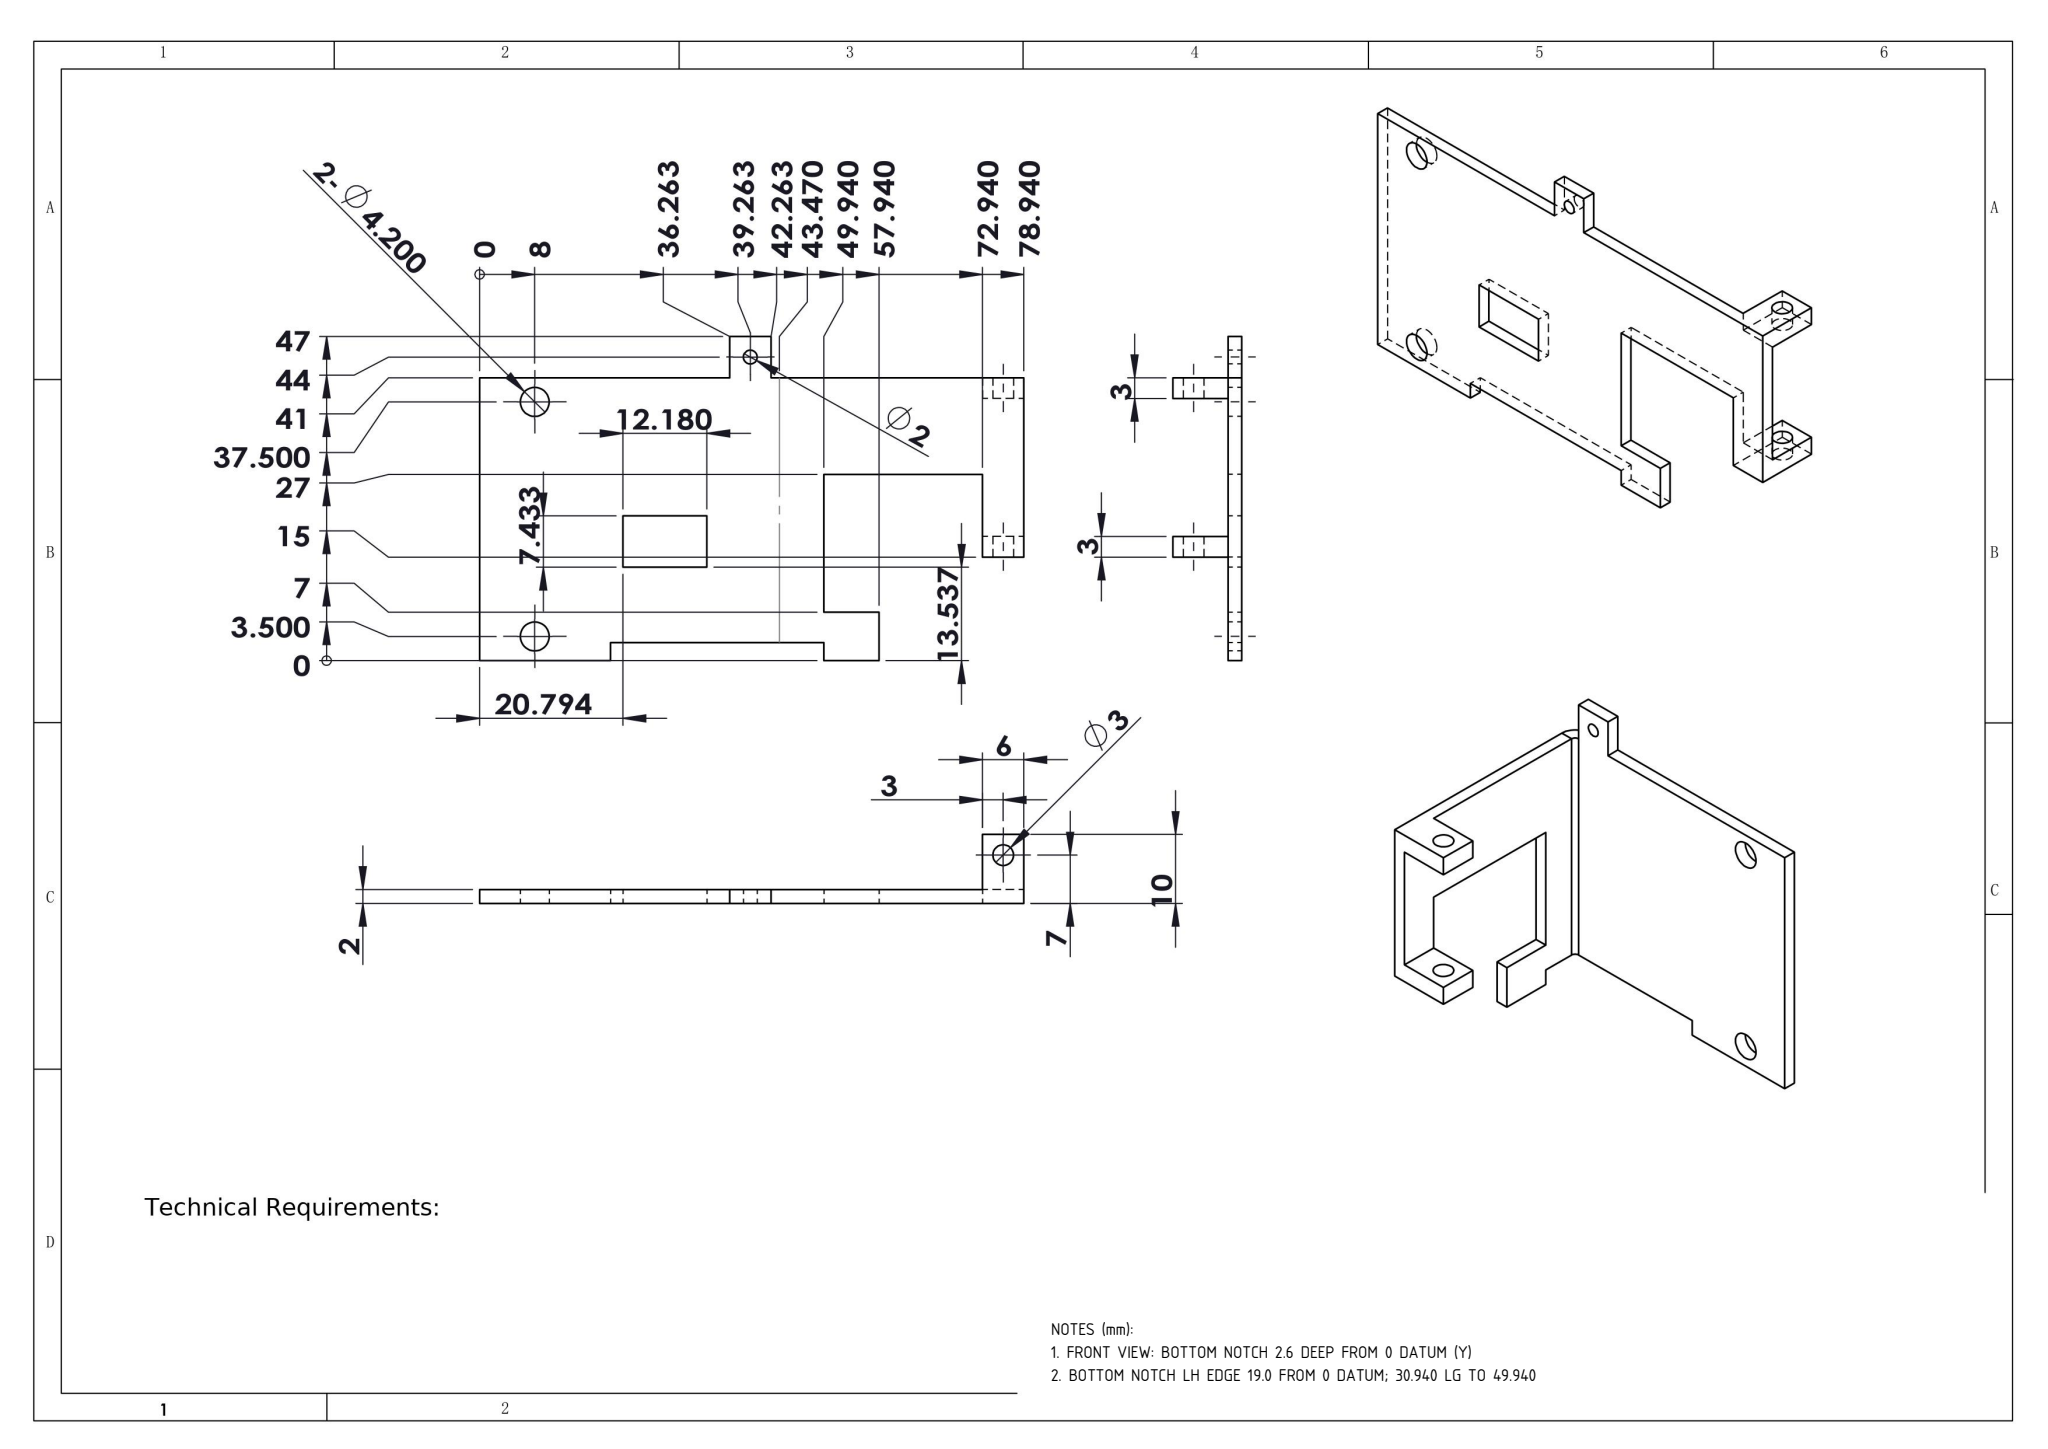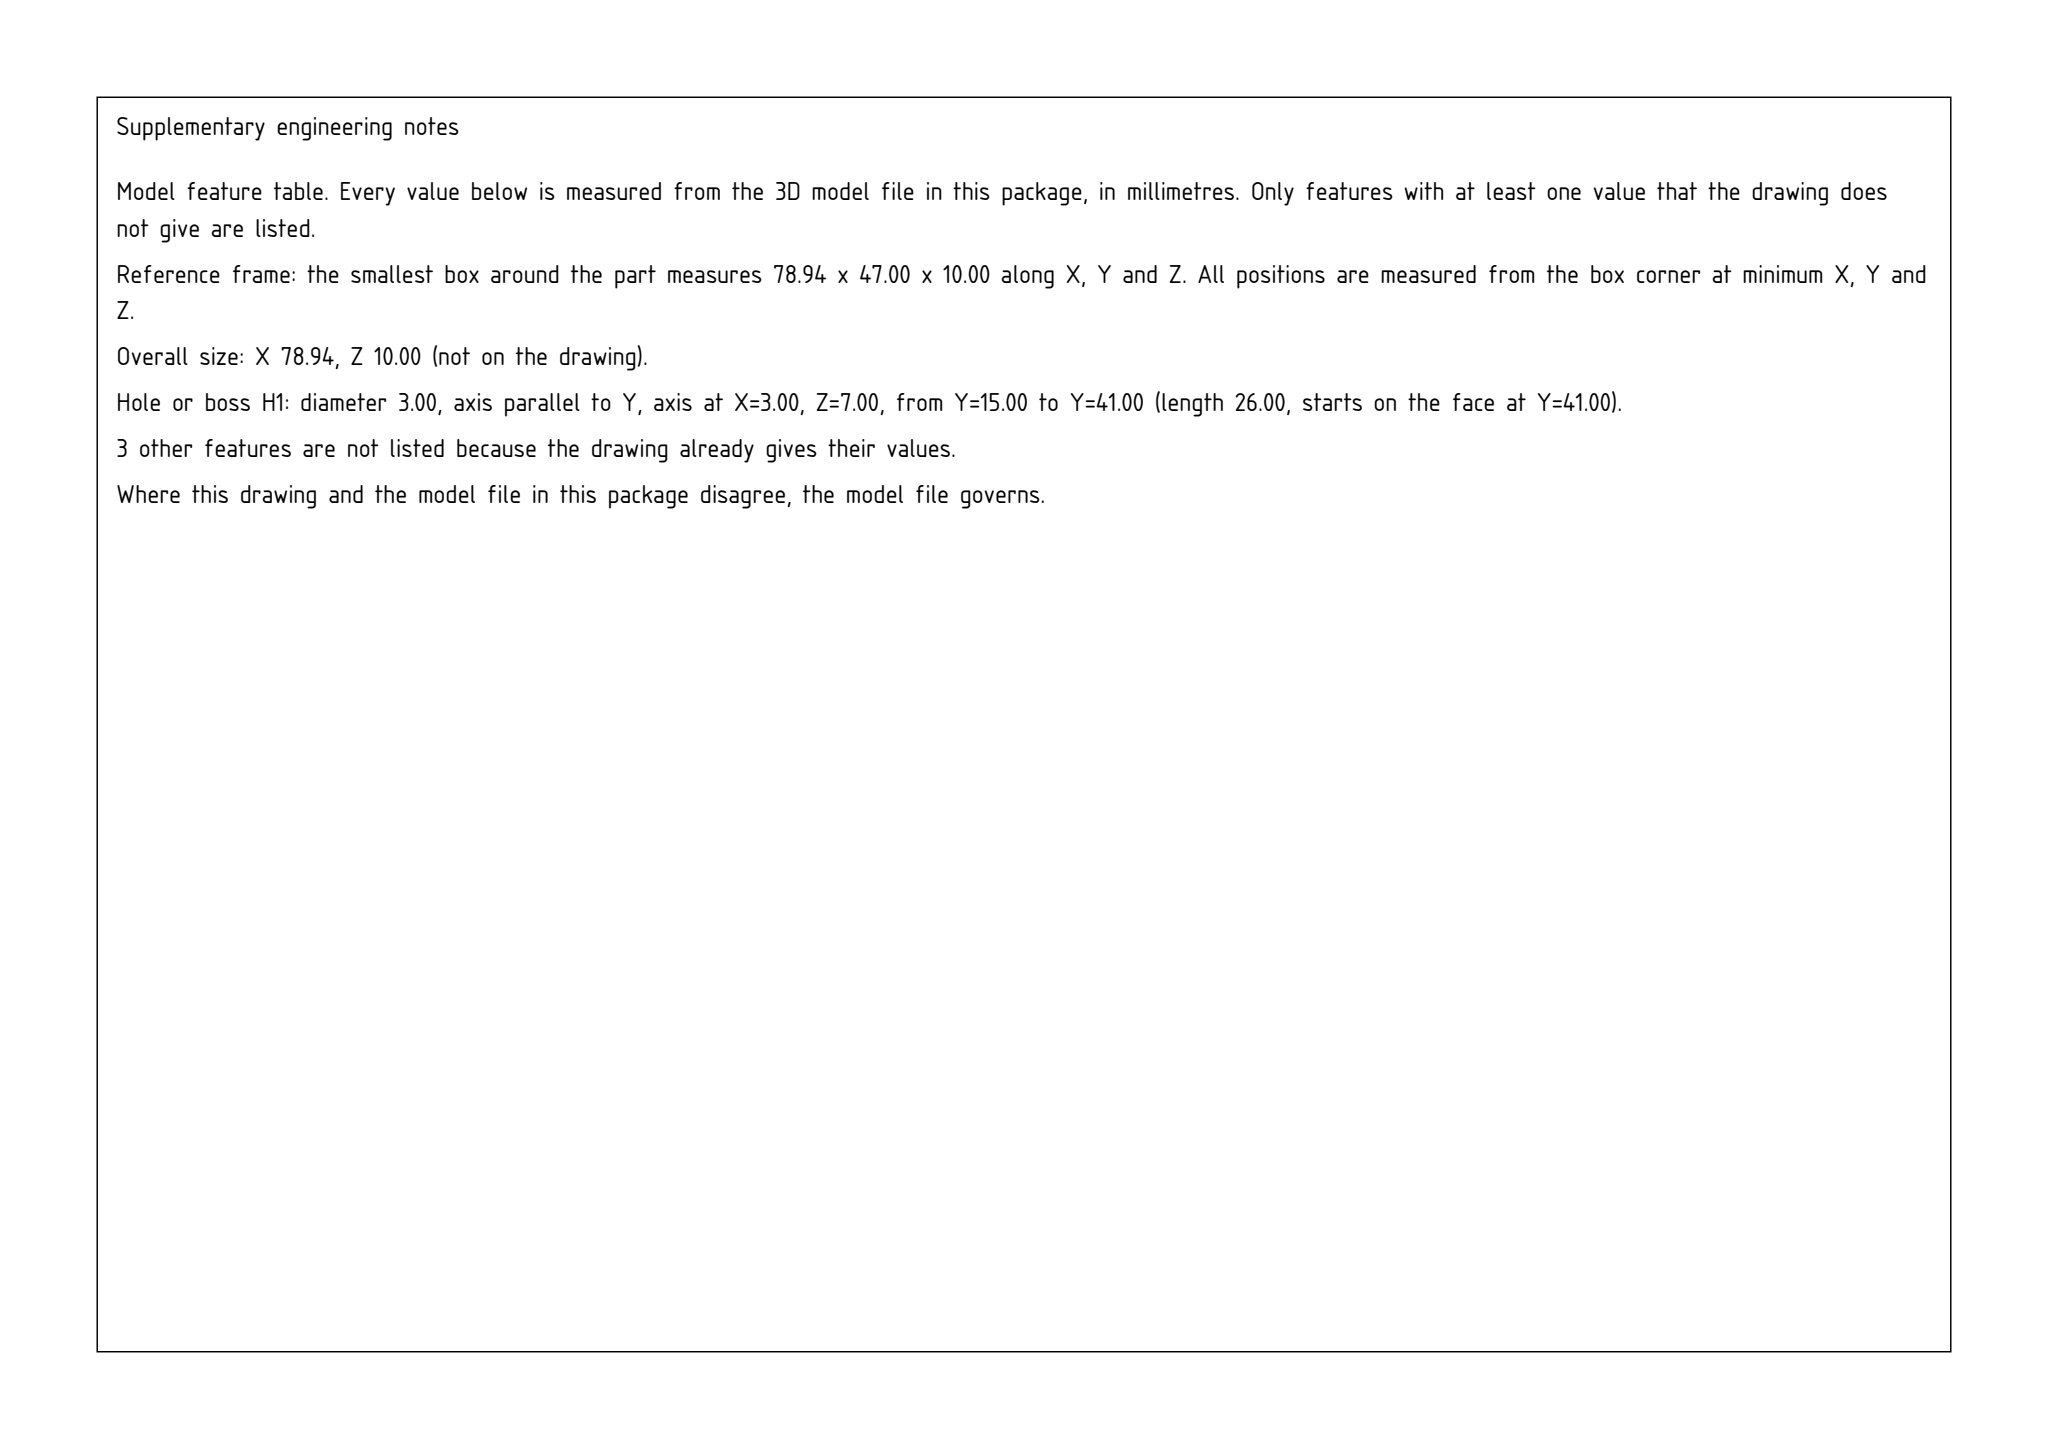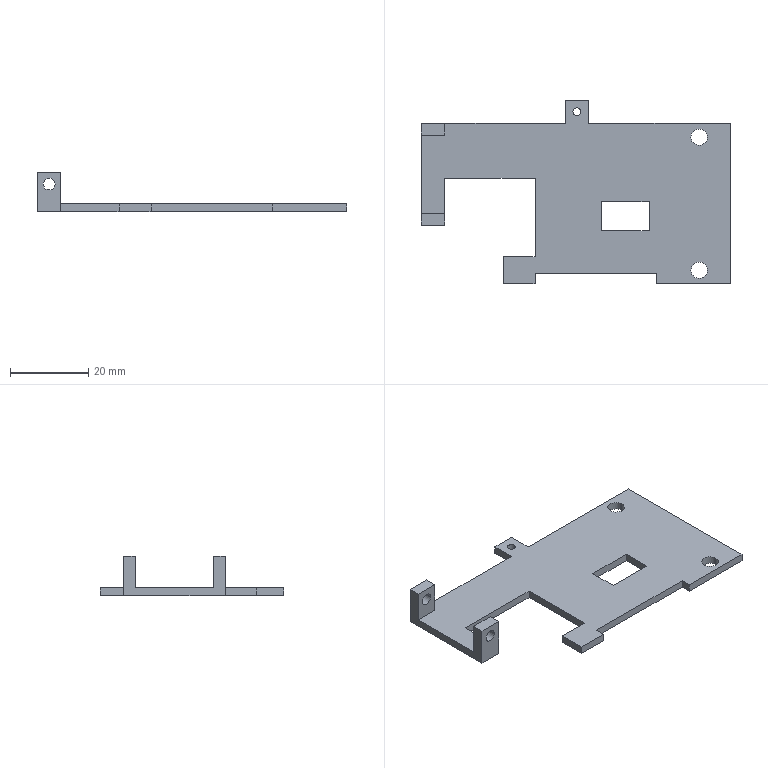Part | SolidWorks | mm | 1 solid | 39 faces | box 78.94 x 47 x 10 mm | volume 5077 mm3 | plane 29 | cylinder 10 | commonest cylinder face diameters 4.2 x4 3 x4 2 x2
Drawing notes:
FRONT VIEW: BOTTOM NOTCH 2.6 DEEP FROM 0 DATUM (Y) | from the solid: Y-normal plane at y=2.6 vs y=0 datum face (bbox min Y)
BOTTOM NOTCH LH EDGE 19.0 FROM 0 DATUM; 30.940 LG TO 49.940 | from the solid: X-normal planes at 59.94 and 29.0; drawing X = 78.94 - STEP X gives 19.0 and 49.940, length 30.94